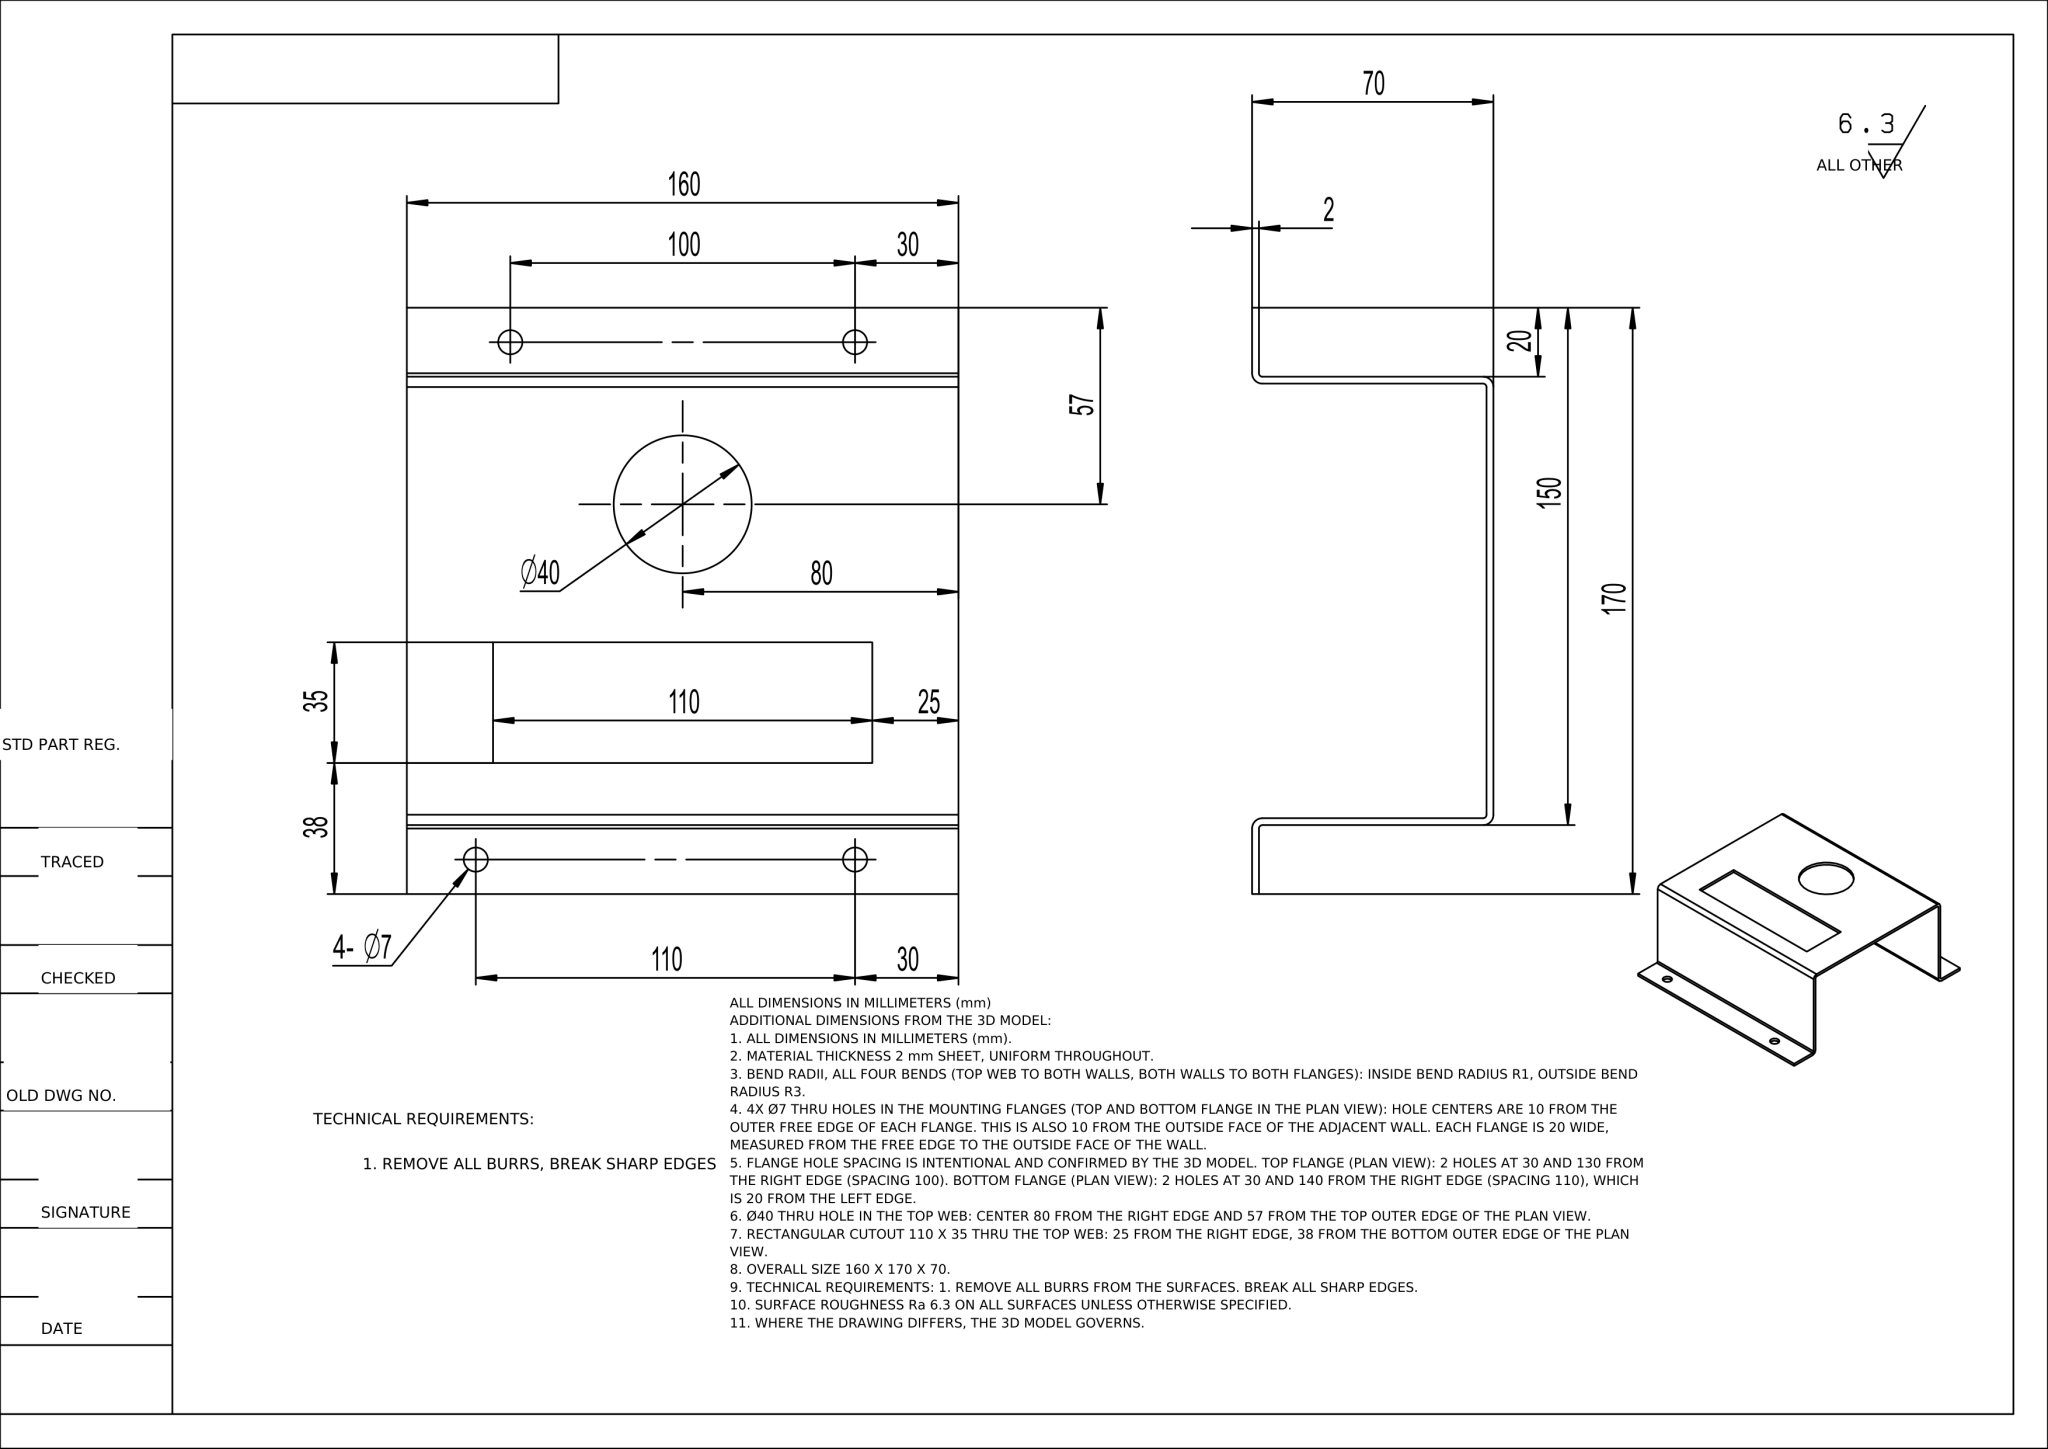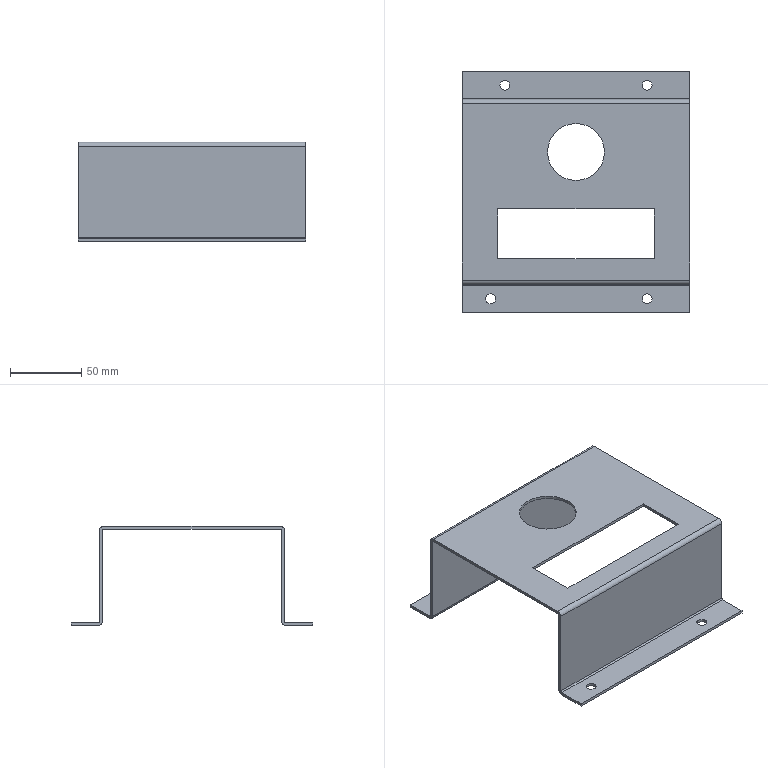Part | NX | mm | 1 solid | 31 faces | box 160 x 170 x 70 mm | volume 86300 mm3 | plane 18 | cylinder 13 | commonest cylinder face diameters 2 x4 6 x4 7 x4 40 x1
STEP:
#1=CARTESIAN_POINT('',(0.,0.,0.));
#2=DIRECTION('',(0.,0.,1.));
#3=DIRECTION('',(1.,0.,0.));
#4=AXIS2_PLACEMENT_3D('',#1,#2,#3);
#5=(LENGTH_UNIT()NAMED_UNIT(*)SI_UNIT(.MILLI.,.METRE.));
#6=UNCERTAINTY_MEASURE_WITH_UNIT(LENGTH_MEASURE(0.00002),#5,'','');
#7=(NAMED_UNIT(*)PLANE_ANGLE_UNIT()SI_UNIT($,.RADIAN.));
#8=PLANE_ANGLE_MEASURE_WITH_UNIT(PLANE_ANGLE_MEASURE(0.01745),#7);
#9=DIMENSIONAL_EXPONENTS(0.,0.,0.,0.,0.,0.,0.);
#10=(CONVERSION_BASED_UNIT('',#8)NAMED_UNIT(#9)PLANE_ANGLE_UNIT());
#11=(NAMED_UNIT(*)SI_UNIT($,.STERADIAN.)SOLID_ANGLE_UNIT());
#12=(GEOMETRIC_REPRESENTATION_CONTEXT(3)GLOBAL_UNCERTAINTY_ASSIGNED_CONTEXT((#6))GLOBAL_UNIT_ASSIGNED_CONTEXT((#5,#10,#11))REPRESENTATION_CONTEXT('',''));
#13=SHAPE_REPRESENTATION('',(#4),#12);
#14=CARTESIAN_POINT('',(25.,38.,68.));
#15=VERTEX_POINT('',#14);
#16=CARTESIAN_POINT('',(135.,38.,68.));
#17=VERTEX_POINT('',#16);
#18=CARTESIAN_POINT('',(25.,38.,68.));
#19=DIRECTION('',(1.,0.,0.));
#20=VECTOR('',#19,1.);
#21=LINE('',#18,#20);
#22=EDGE_CURVE('',#15,#17,#21,.T.);
#23=ORIENTED_EDGE('',*,*,#22,.F.);
#24=CARTESIAN_POINT('',(25.,73.,68.));
#25=VERTEX_POINT('',#24);
#26=CARTESIAN_POINT('',(25.,73.,68.));
#27=DIRECTION('',(0.,-1.,0.));
#28=VECTOR('',#27,1.);
#29=LINE('',#26,#28);
#30=EDGE_CURVE('',#25,#15,#29,.T.);
#31=ORIENTED_EDGE('',*,*,#30,.F.);
#32=CARTESIAN_POINT('',(135.,73.,68.));
#33=VERTEX_POINT('',#32);
#34=CARTESIAN_POINT('',(135.,73.,68.));
#35=DIRECTION('',(-1.,-0.,0.));
#36=VECTOR('',#35,1.);
#37=LINE('',#34,#36);
#38=EDGE_CURVE('',#33,#25,#37,.T.);
#39=ORIENTED_EDGE('',*,*,#38,.F.);
#40=CARTESIAN_POINT('',(135.,38.,68.));
#41=DIRECTION('',(0.,1.,0.));
#42=VECTOR('',#41,1.);
#43=LINE('',#40,#42);
#44=EDGE_CURVE('',#17,#33,#43,.T.);
#45=ORIENTED_EDGE('',*,*,#44,.F.);
#46=EDGE_LOOP('',(#23,#31,#39,#45));
#47=FACE_BOUND('',#46,.T.);
#48=CARTESIAN_POINT('',(160.,23.,68.));
#49=VERTEX_POINT('',#48);
#50=CARTESIAN_POINT('',(160.,147.,68.));
#51=VERTEX_POINT('',#50);
#52=CARTESIAN_POINT('',(160.,20.,68.));
#53=DIRECTION('',(0.,1.,0.));
#54=VECTOR('',#53,1.);
#55=LINE('',#52,#54);
#56=EDGE_CURVE('',#49,#51,#55,.T.);
#57=ORIENTED_EDGE('',*,*,#56,.T.);
#58=CARTESIAN_POINT('',(0.,147.,68.));
#59=VERTEX_POINT('',#58);
#60=CARTESIAN_POINT('',(0.,147.,68.));
#61=DIRECTION('',(1.,0.,0.));
#62=VECTOR('',#61,1.);
#63=LINE('',#60,#62);
#64=EDGE_CURVE('',#59,#51,#63,.T.);
#65=ORIENTED_EDGE('',*,*,#64,.F.);
#66=CARTESIAN_POINT('',(0.,23.,68.));
#67=VERTEX_POINT('',#66);
#68=CARTESIAN_POINT('',(0.,20.,68.));
#69=DIRECTION('',(0.,1.,0.));
#70=VECTOR('',#69,1.);
#71=LINE('',#68,#70);
#72=EDGE_CURVE('',#67,#59,#71,.T.);
#73=ORIENTED_EDGE('',*,*,#72,.F.);
#74=CARTESIAN_POINT('',(0.,23.,68.));
#75=DIRECTION('',(1.,0.,0.));
#76=VECTOR('',#75,1.);
#77=LINE('',#74,#76);
#78=EDGE_CURVE('',#67,#49,#77,.T.);
#79=ORIENTED_EDGE('',*,*,#78,.T.);
#80=EDGE_LOOP('',(#57,#65,#73,#79));
#81=FACE_BOUND('',#80,.T.);
#82=CARTESIAN_POINT('',(60.,113.,68.));
#83=VERTEX_POINT('',#82);
#84=CARTESIAN_POINT('',(80.,113.,68.));
#85=DIRECTION('',(0.,0.,1.));
#86=DIRECTION('',(-1.,0.,0.));
#87=AXIS2_PLACEMENT_3D('',#84,#85,#86);
#88=CIRCLE('',#87,20.);
#89=EDGE_CURVE('',#83,#83,#88,.T.);
#90=ORIENTED_EDGE('',*,*,#89,.F.);
#91=EDGE_LOOP('',(#90));
#92=FACE_BOUND('',#91,.T.);
#93=CARTESIAN_POINT('',(0.,20.,68.));
#94=DIRECTION('',(0.,0.,-1.));
#95=DIRECTION('',(-1.,0.,0.));
#96=AXIS2_PLACEMENT_3D('',#93,#94,#95);
#97=PLANE('',#96);
#98=ADVANCED_FACE('',(#47,#81,#92),#97,.F.);
#99=CARTESIAN_POINT('',(160.,170.,-2.));
#100=VERTEX_POINT('',#99);
#101=CARTESIAN_POINT('',(160.,170.,0.));
#102=VERTEX_POINT('',#101);
#103=CARTESIAN_POINT('',(160.,170.,0.));
#104=DIRECTION('',(0.,0.,1.));
#105=VECTOR('',#104,1.);
#106=LINE('',#103,#105);
#107=EDGE_CURVE('',#100,#102,#106,.T.);
#108=ORIENTED_EDGE('',*,*,#107,.F.);
#109=CARTESIAN_POINT('',(0.,170.,-2.));
#110=VERTEX_POINT('',#109);
#111=CARTESIAN_POINT('',(0.,170.,-2.));
#112=DIRECTION('',(1.,0.,0.));
#113=VECTOR('',#112,1.);
#114=LINE('',#111,#113);
#115=EDGE_CURVE('',#110,#100,#114,.T.);
#116=ORIENTED_EDGE('',*,*,#115,.F.);
#117=CARTESIAN_POINT('',(0.,170.,0.));
#118=VERTEX_POINT('',#117);
#119=CARTESIAN_POINT('',(0.,170.,0.));
#120=DIRECTION('',(0.,0.,1.));
#121=VECTOR('',#120,1.);
#122=LINE('',#119,#121);
#123=EDGE_CURVE('',#110,#118,#122,.T.);
#124=ORIENTED_EDGE('',*,*,#123,.T.);
#125=CARTESIAN_POINT('',(0.,170.,0.));
#126=DIRECTION('',(1.,0.,0.));
#127=VECTOR('',#126,1.);
#128=LINE('',#125,#127);
#129=EDGE_CURVE('',#118,#102,#128,.T.);
#130=ORIENTED_EDGE('',*,*,#129,.T.);
#131=EDGE_LOOP('',(#108,#116,#124,#130));
#132=FACE_OUTER_BOUND('',#131,.T.);
#133=CARTESIAN_POINT('',(0.,170.,0.));
#134=DIRECTION('',(0.,1.,0.));
#135=DIRECTION('',(1.,0.,0.));
#136=AXIS2_PLACEMENT_3D('',#133,#134,#135);
#137=PLANE('',#136);
#138=ADVANCED_FACE('',(#132),#137,.T.);
#139=CARTESIAN_POINT('',(0.,0.,0.));
#140=VERTEX_POINT('',#139);
#141=CARTESIAN_POINT('',(0.,19.,0.));
#142=VERTEX_POINT('',#141);
#143=CARTESIAN_POINT('',(0.,0.,0.));
#144=DIRECTION('',(0.,1.,0.));
#145=VECTOR('',#144,1.);
#146=LINE('',#143,#145);
#147=EDGE_CURVE('',#140,#142,#146,.T.);
#148=ORIENTED_EDGE('',*,*,#147,.T.);
#149=CARTESIAN_POINT('',(0.,20.,1.));
#150=VERTEX_POINT('',#149);
#151=CARTESIAN_POINT('',(0.,19.,1.));
#152=DIRECTION('',(1.,0.,0.));
#153=DIRECTION('',(0.,0.,1.));
#154=AXIS2_PLACEMENT_3D('',#151,#152,#153);
#155=CIRCLE('',#154,1.);
#156=EDGE_CURVE('',#142,#150,#155,.T.);
#157=ORIENTED_EDGE('',*,*,#156,.T.);
#158=CARTESIAN_POINT('',(0.,20.,65.));
#159=VERTEX_POINT('',#158);
#160=CARTESIAN_POINT('',(0.,20.,0.));
#161=DIRECTION('',(0.,0.,1.));
#162=VECTOR('',#161,1.);
#163=LINE('',#160,#162);
#164=EDGE_CURVE('',#150,#159,#163,.T.);
#165=ORIENTED_EDGE('',*,*,#164,.T.);
#166=CARTESIAN_POINT('',(0.,23.,65.));
#167=DIRECTION('',(-1.,0.,0.));
#168=DIRECTION('',(0.,0.,-1.));
#169=AXIS2_PLACEMENT_3D('',#166,#167,#168);
#170=CIRCLE('',#169,3.);
#171=EDGE_CURVE('',#159,#67,#170,.T.);
#172=ORIENTED_EDGE('',*,*,#171,.T.);
#173=ORIENTED_EDGE('',*,*,#72,.T.);
#174=CARTESIAN_POINT('',(0.,150.,65.));
#175=VERTEX_POINT('',#174);
#176=CARTESIAN_POINT('',(0.,147.,65.));
#177=DIRECTION('',(-1.,0.,0.));
#178=DIRECTION('',(0.,0.,-1.));
#179=AXIS2_PLACEMENT_3D('',#176,#177,#178);
#180=CIRCLE('',#179,3.);
#181=EDGE_CURVE('',#59,#175,#180,.T.);
#182=ORIENTED_EDGE('',*,*,#181,.T.);
#183=CARTESIAN_POINT('',(0.,150.,1.));
#184=VERTEX_POINT('',#183);
#185=CARTESIAN_POINT('',(0.,150.,68.));
#186=DIRECTION('',(0.,0.,-1.));
#187=VECTOR('',#186,1.);
#188=LINE('',#185,#187);
#189=EDGE_CURVE('',#175,#184,#188,.T.);
#190=ORIENTED_EDGE('',*,*,#189,.T.);
#191=CARTESIAN_POINT('',(0.,151.,0.));
#192=VERTEX_POINT('',#191);
#193=CARTESIAN_POINT('',(0.,151.,1.));
#194=DIRECTION('',(1.,0.,0.));
#195=DIRECTION('',(0.,0.,1.));
#196=AXIS2_PLACEMENT_3D('',#193,#194,#195);
#197=CIRCLE('',#196,1.);
#198=EDGE_CURVE('',#184,#192,#197,.T.);
#199=ORIENTED_EDGE('',*,*,#198,.T.);
#200=CARTESIAN_POINT('',(0.,150.,0.));
#201=DIRECTION('',(0.,1.,0.));
#202=VECTOR('',#201,1.);
#203=LINE('',#200,#202);
#204=EDGE_CURVE('',#192,#118,#203,.T.);
#205=ORIENTED_EDGE('',*,*,#204,.T.);
#206=ORIENTED_EDGE('',*,*,#123,.F.);
#207=CARTESIAN_POINT('',(0.,151.,-2.));
#208=VERTEX_POINT('',#207);
#209=CARTESIAN_POINT('',(0.,150.,-2.));
#210=DIRECTION('',(0.,1.,0.));
#211=VECTOR('',#210,1.);
#212=LINE('',#209,#211);
#213=EDGE_CURVE('',#208,#110,#212,.T.);
#214=ORIENTED_EDGE('',*,*,#213,.F.);
#215=CARTESIAN_POINT('',(0.,148.,1.));
#216=VERTEX_POINT('',#215);
#217=CARTESIAN_POINT('',(0.,151.,1.));
#218=DIRECTION('',(1.,0.,0.));
#219=DIRECTION('',(0.,0.,-1.));
#220=AXIS2_PLACEMENT_3D('',#217,#218,#219);
#221=CIRCLE('',#220,3.);
#222=EDGE_CURVE('',#216,#208,#221,.T.);
#223=ORIENTED_EDGE('',*,*,#222,.F.);
#224=CARTESIAN_POINT('',(0.,148.,65.));
#225=VERTEX_POINT('',#224);
#226=CARTESIAN_POINT('',(0.,148.,68.));
#227=DIRECTION('',(0.,0.,-1.));
#228=VECTOR('',#227,1.);
#229=LINE('',#226,#228);
#230=EDGE_CURVE('',#225,#216,#229,.T.);
#231=ORIENTED_EDGE('',*,*,#230,.F.);
#232=CARTESIAN_POINT('',(0.,147.,66.));
#233=VERTEX_POINT('',#232);
#234=CARTESIAN_POINT('',(0.,147.,65.));
#235=DIRECTION('',(-1.,0.,0.));
#236=DIRECTION('',(0.,0.,-1.));
#237=AXIS2_PLACEMENT_3D('',#234,#235,#236);
#238=CIRCLE('',#237,1.);
#239=EDGE_CURVE('',#233,#225,#238,.T.);
#240=ORIENTED_EDGE('',*,*,#239,.F.);
#241=CARTESIAN_POINT('',(0.,23.,66.));
#242=VERTEX_POINT('',#241);
#243=CARTESIAN_POINT('',(0.,20.,66.));
#244=DIRECTION('',(0.,1.,0.));
#245=VECTOR('',#244,1.);
#246=LINE('',#243,#245);
#247=EDGE_CURVE('',#242,#233,#246,.T.);
#248=ORIENTED_EDGE('',*,*,#247,.F.);
#249=CARTESIAN_POINT('',(0.,22.,65.));
#250=VERTEX_POINT('',#249);
#251=CARTESIAN_POINT('',(0.,23.,65.));
#252=DIRECTION('',(-1.,0.,0.));
#253=DIRECTION('',(0.,0.,-1.));
#254=AXIS2_PLACEMENT_3D('',#251,#252,#253);
#255=CIRCLE('',#254,1.);
#256=EDGE_CURVE('',#250,#242,#255,.T.);
#257=ORIENTED_EDGE('',*,*,#256,.F.);
#258=CARTESIAN_POINT('',(0.,22.,1.));
#259=VERTEX_POINT('',#258);
#260=CARTESIAN_POINT('',(0.,22.,-0.));
#261=DIRECTION('',(0.,0.,1.));
#262=VECTOR('',#261,1.);
#263=LINE('',#260,#262);
#264=EDGE_CURVE('',#259,#250,#263,.T.);
#265=ORIENTED_EDGE('',*,*,#264,.F.);
#266=CARTESIAN_POINT('',(0.,19.,-2.));
#267=VERTEX_POINT('',#266);
#268=CARTESIAN_POINT('',(0.,19.,1.));
#269=DIRECTION('',(1.,0.,0.));
#270=DIRECTION('',(0.,0.,-1.));
#271=AXIS2_PLACEMENT_3D('',#268,#269,#270);
#272=CIRCLE('',#271,3.);
#273=EDGE_CURVE('',#267,#259,#272,.T.);
#274=ORIENTED_EDGE('',*,*,#273,.F.);
#275=CARTESIAN_POINT('',(0.,0.,-2.));
#276=VERTEX_POINT('',#275);
#277=CARTESIAN_POINT('',(0.,0.,-2.));
#278=DIRECTION('',(0.,1.,0.));
#279=VECTOR('',#278,1.);
#280=LINE('',#277,#279);
#281=EDGE_CURVE('',#276,#267,#280,.T.);
#282=ORIENTED_EDGE('',*,*,#281,.F.);
#283=CARTESIAN_POINT('',(0.,0.,0.));
#284=DIRECTION('',(0.,0.,1.));
#285=VECTOR('',#284,1.);
#286=LINE('',#283,#285);
#287=EDGE_CURVE('',#276,#140,#286,.T.);
#288=ORIENTED_EDGE('',*,*,#287,.T.);
#289=EDGE_LOOP('',(#148,#157,#165,#172,#173,#182,#190,#199,#205,#206,#214,#223,#231,#240,#248,#257,#265,#274,#282,#288));
#290=FACE_OUTER_BOUND('',#289,.T.);
#291=CARTESIAN_POINT('',(0.,0.,0.));
#292=DIRECTION('',(-1.,0.,0.));
#293=DIRECTION('',(0.,1.,0.));
#294=AXIS2_PLACEMENT_3D('',#291,#292,#293);
#295=PLANE('',#294);
#296=ADVANCED_FACE('',(#290),#295,.T.);
#297=ORIENTED_EDGE('',*,*,#287,.F.);
#298=CARTESIAN_POINT('',(160.,0.,-2.));
#299=VERTEX_POINT('',#298);
#300=CARTESIAN_POINT('',(0.,0.,-2.));
#301=DIRECTION('',(1.,0.,0.));
#302=VECTOR('',#301,1.);
#303=LINE('',#300,#302);
#304=EDGE_CURVE('',#276,#299,#303,.T.);
#305=ORIENTED_EDGE('',*,*,#304,.T.);
#306=CARTESIAN_POINT('',(160.,0.,0.));
#307=VERTEX_POINT('',#306);
#308=CARTESIAN_POINT('',(160.,0.,0.));
#309=DIRECTION('',(0.,0.,1.));
#310=VECTOR('',#309,1.);
#311=LINE('',#308,#310);
#312=EDGE_CURVE('',#299,#307,#311,.T.);
#313=ORIENTED_EDGE('',*,*,#312,.T.);
#314=CARTESIAN_POINT('',(0.,0.,0.));
#315=DIRECTION('',(1.,0.,0.));
#316=VECTOR('',#315,1.);
#317=LINE('',#314,#316);
#318=EDGE_CURVE('',#140,#307,#317,.T.);
#319=ORIENTED_EDGE('',*,*,#318,.F.);
#320=EDGE_LOOP('',(#297,#305,#313,#319));
#321=FACE_OUTER_BOUND('',#320,.T.);
#322=CARTESIAN_POINT('',(0.,0.,0.));
#323=DIRECTION('',(0.,1.,0.));
#324=DIRECTION('',(1.,0.,0.));
#325=AXIS2_PLACEMENT_3D('',#322,#323,#324);
#326=PLANE('',#325);
#327=ADVANCED_FACE('',(#321),#326,.F.);
#328=CARTESIAN_POINT('',(160.,19.,-2.));
#329=VERTEX_POINT('',#328);
#330=CARTESIAN_POINT('',(160.,22.,1.));
#331=VERTEX_POINT('',#330);
#332=CARTESIAN_POINT('',(160.,19.,1.));
#333=DIRECTION('',(1.,0.,0.));
#334=DIRECTION('',(0.,0.,-1.));
#335=AXIS2_PLACEMENT_3D('',#332,#333,#334);
#336=CIRCLE('',#335,3.);
#337=EDGE_CURVE('',#329,#331,#336,.T.);
#338=ORIENTED_EDGE('',*,*,#337,.T.);
#339=CARTESIAN_POINT('',(160.,22.,65.));
#340=VERTEX_POINT('',#339);
#341=CARTESIAN_POINT('',(160.,22.,-0.));
#342=DIRECTION('',(0.,0.,1.));
#343=VECTOR('',#342,1.);
#344=LINE('',#341,#343);
#345=EDGE_CURVE('',#331,#340,#344,.T.);
#346=ORIENTED_EDGE('',*,*,#345,.T.);
#347=CARTESIAN_POINT('',(160.,23.,66.));
#348=VERTEX_POINT('',#347);
#349=CARTESIAN_POINT('',(160.,23.,65.));
#350=DIRECTION('',(-1.,0.,0.));
#351=DIRECTION('',(0.,0.,-1.));
#352=AXIS2_PLACEMENT_3D('',#349,#350,#351);
#353=CIRCLE('',#352,1.);
#354=EDGE_CURVE('',#340,#348,#353,.T.);
#355=ORIENTED_EDGE('',*,*,#354,.T.);
#356=CARTESIAN_POINT('',(160.,147.,66.));
#357=VERTEX_POINT('',#356);
#358=CARTESIAN_POINT('',(160.,20.,66.));
#359=DIRECTION('',(0.,1.,0.));
#360=VECTOR('',#359,1.);
#361=LINE('',#358,#360);
#362=EDGE_CURVE('',#348,#357,#361,.T.);
#363=ORIENTED_EDGE('',*,*,#362,.T.);
#364=CARTESIAN_POINT('',(160.,148.,65.));
#365=VERTEX_POINT('',#364);
#366=CARTESIAN_POINT('',(160.,147.,65.));
#367=DIRECTION('',(-1.,0.,0.));
#368=DIRECTION('',(0.,0.,-1.));
#369=AXIS2_PLACEMENT_3D('',#366,#367,#368);
#370=CIRCLE('',#369,1.);
#371=EDGE_CURVE('',#357,#365,#370,.T.);
#372=ORIENTED_EDGE('',*,*,#371,.T.);
#373=CARTESIAN_POINT('',(160.,148.,1.));
#374=VERTEX_POINT('',#373);
#375=CARTESIAN_POINT('',(160.,148.,68.));
#376=DIRECTION('',(0.,0.,-1.));
#377=VECTOR('',#376,1.);
#378=LINE('',#375,#377);
#379=EDGE_CURVE('',#365,#374,#378,.T.);
#380=ORIENTED_EDGE('',*,*,#379,.T.);
#381=CARTESIAN_POINT('',(160.,151.,-2.));
#382=VERTEX_POINT('',#381);
#383=CARTESIAN_POINT('',(160.,151.,1.));
#384=DIRECTION('',(1.,0.,0.));
#385=DIRECTION('',(0.,0.,-1.));
#386=AXIS2_PLACEMENT_3D('',#383,#384,#385);
#387=CIRCLE('',#386,3.);
#388=EDGE_CURVE('',#374,#382,#387,.T.);
#389=ORIENTED_EDGE('',*,*,#388,.T.);
#390=CARTESIAN_POINT('',(160.,150.,-2.));
#391=DIRECTION('',(0.,1.,0.));
#392=VECTOR('',#391,1.);
#393=LINE('',#390,#392);
#394=EDGE_CURVE('',#382,#100,#393,.T.);
#395=ORIENTED_EDGE('',*,*,#394,.T.);
#396=ORIENTED_EDGE('',*,*,#107,.T.);
#397=CARTESIAN_POINT('',(160.,151.,0.));
#398=VERTEX_POINT('',#397);
#399=CARTESIAN_POINT('',(160.,150.,0.));
#400=DIRECTION('',(0.,1.,0.));
#401=VECTOR('',#400,1.);
#402=LINE('',#399,#401);
#403=EDGE_CURVE('',#398,#102,#402,.T.);
#404=ORIENTED_EDGE('',*,*,#403,.F.);
#405=CARTESIAN_POINT('',(160.,150.,1.));
#406=VERTEX_POINT('',#405);
#407=CARTESIAN_POINT('',(160.,151.,1.));
#408=DIRECTION('',(1.,0.,0.));
#409=DIRECTION('',(0.,0.,1.));
#410=AXIS2_PLACEMENT_3D('',#407,#408,#409);
#411=CIRCLE('',#410,1.);
#412=EDGE_CURVE('',#406,#398,#411,.T.);
#413=ORIENTED_EDGE('',*,*,#412,.F.);
#414=CARTESIAN_POINT('',(160.,150.,65.));
#415=VERTEX_POINT('',#414);
#416=CARTESIAN_POINT('',(160.,150.,68.));
#417=DIRECTION('',(0.,0.,-1.));
#418=VECTOR('',#417,1.);
#419=LINE('',#416,#418);
#420=EDGE_CURVE('',#415,#406,#419,.T.);
#421=ORIENTED_EDGE('',*,*,#420,.F.);
#422=CARTESIAN_POINT('',(160.,147.,65.));
#423=DIRECTION('',(-1.,0.,0.));
#424=DIRECTION('',(0.,0.,-1.));
#425=AXIS2_PLACEMENT_3D('',#422,#423,#424);
#426=CIRCLE('',#425,3.);
#427=EDGE_CURVE('',#51,#415,#426,.T.);
#428=ORIENTED_EDGE('',*,*,#427,.F.);
#429=ORIENTED_EDGE('',*,*,#56,.F.);
#430=CARTESIAN_POINT('',(160.,20.,65.));
#431=VERTEX_POINT('',#430);
#432=CARTESIAN_POINT('',(160.,23.,65.));
#433=DIRECTION('',(-1.,0.,0.));
#434=DIRECTION('',(0.,0.,-1.));
#435=AXIS2_PLACEMENT_3D('',#432,#433,#434);
#436=CIRCLE('',#435,3.);
#437=EDGE_CURVE('',#431,#49,#436,.T.);
#438=ORIENTED_EDGE('',*,*,#437,.F.);
#439=CARTESIAN_POINT('',(160.,20.,1.));
#440=VERTEX_POINT('',#439);
#441=CARTESIAN_POINT('',(160.,20.,0.));
#442=DIRECTION('',(0.,0.,1.));
#443=VECTOR('',#442,1.);
#444=LINE('',#441,#443);
#445=EDGE_CURVE('',#440,#431,#444,.T.);
#446=ORIENTED_EDGE('',*,*,#445,.F.);
#447=CARTESIAN_POINT('',(160.,19.,0.));
#448=VERTEX_POINT('',#447);
#449=CARTESIAN_POINT('',(160.,19.,1.));
#450=DIRECTION('',(1.,0.,0.));
#451=DIRECTION('',(0.,0.,1.));
#452=AXIS2_PLACEMENT_3D('',#449,#450,#451);
#453=CIRCLE('',#452,1.);
#454=EDGE_CURVE('',#448,#440,#453,.T.);
#455=ORIENTED_EDGE('',*,*,#454,.F.);
#456=CARTESIAN_POINT('',(160.,0.,0.));
#457=DIRECTION('',(0.,1.,0.));
#458=VECTOR('',#457,1.);
#459=LINE('',#456,#458);
#460=EDGE_CURVE('',#307,#448,#459,.T.);
#461=ORIENTED_EDGE('',*,*,#460,.F.);
#462=ORIENTED_EDGE('',*,*,#312,.F.);
#463=CARTESIAN_POINT('',(160.,0.,-2.));
#464=DIRECTION('',(0.,1.,0.));
#465=VECTOR('',#464,1.);
#466=LINE('',#463,#465);
#467=EDGE_CURVE('',#299,#329,#466,.T.);
#468=ORIENTED_EDGE('',*,*,#467,.T.);
#469=EDGE_LOOP('',(#338,#346,#355,#363,#372,#380,#389,#395,#396,#404,#413,#421,#428,#429,#438,#446,#455,#461,#462,#468));
#470=FACE_OUTER_BOUND('',#469,.T.);
#471=CARTESIAN_POINT('',(160.,19.,1.));
#472=DIRECTION('',(1.,0.,0.));
#473=DIRECTION('',(0.,0.,-1.));
#474=AXIS2_PLACEMENT_3D('',#471,#472,#473);
#475=PLANE('',#474);
#476=ADVANCED_FACE('',(#470),#475,.T.);
#477=CARTESIAN_POINT('',(126.5,10.,0.));
#478=VERTEX_POINT('',#477);
#479=CARTESIAN_POINT('',(130.,10.,0.));
#480=DIRECTION('',(0.,0.,-1.));
#481=DIRECTION('',(-1.,0.,0.));
#482=AXIS2_PLACEMENT_3D('',#479,#480,#481);
#483=CIRCLE('',#482,3.5);
#484=EDGE_CURVE('',#478,#478,#483,.T.);
#485=ORIENTED_EDGE('',*,*,#484,.T.);
#486=EDGE_LOOP('',(#485));
#487=FACE_BOUND('',#486,.T.);
#488=CARTESIAN_POINT('',(16.5,10.,0.));
#489=VERTEX_POINT('',#488);
#490=CARTESIAN_POINT('',(20.,10.,0.));
#491=DIRECTION('',(0.,0.,-1.));
#492=DIRECTION('',(-1.,0.,0.));
#493=AXIS2_PLACEMENT_3D('',#490,#491,#492);
#494=CIRCLE('',#493,3.5);
#495=EDGE_CURVE('',#489,#489,#494,.T.);
#496=ORIENTED_EDGE('',*,*,#495,.T.);
#497=EDGE_LOOP('',(#496));
#498=FACE_BOUND('',#497,.T.);
#499=ORIENTED_EDGE('',*,*,#460,.T.);
#500=CARTESIAN_POINT('',(0.,19.,0.));
#501=DIRECTION('',(1.,0.,0.));
#502=VECTOR('',#501,1.);
#503=LINE('',#500,#502);
#504=EDGE_CURVE('',#142,#448,#503,.T.);
#505=ORIENTED_EDGE('',*,*,#504,.F.);
#506=ORIENTED_EDGE('',*,*,#147,.F.);
#507=ORIENTED_EDGE('',*,*,#318,.T.);
#508=EDGE_LOOP('',(#499,#505,#506,#507));
#509=FACE_BOUND('',#508,.T.);
#510=CARTESIAN_POINT('',(0.,0.,0.));
#511=DIRECTION('',(0.,0.,-1.));
#512=DIRECTION('',(-1.,0.,0.));
#513=AXIS2_PLACEMENT_3D('',#510,#511,#512);
#514=PLANE('',#513);
#515=ADVANCED_FACE('',(#487,#498,#509),#514,.F.);
#516=ORIENTED_EDGE('',*,*,#454,.T.);
#517=CARTESIAN_POINT('',(0.,20.,1.));
#518=DIRECTION('',(1.,0.,0.));
#519=VECTOR('',#518,1.);
#520=LINE('',#517,#519);
#521=EDGE_CURVE('',#150,#440,#520,.T.);
#522=ORIENTED_EDGE('',*,*,#521,.F.);
#523=ORIENTED_EDGE('',*,*,#156,.F.);
#524=ORIENTED_EDGE('',*,*,#504,.T.);
#525=EDGE_LOOP('',(#516,#522,#523,#524));
#526=FACE_OUTER_BOUND('',#525,.T.);
#527=CARTESIAN_POINT('',(0.,19.,1.));
#528=DIRECTION('',(1.,0.,0.));
#529=DIRECTION('',(0.,0.,-1.));
#530=AXIS2_PLACEMENT_3D('',#527,#528,#529);
#531=CYLINDRICAL_SURFACE('',#530,1.);
#532=ADVANCED_FACE('',(#526),#531,.F.);
#533=ORIENTED_EDGE('',*,*,#445,.T.);
#534=CARTESIAN_POINT('',(0.,20.,65.));
#535=DIRECTION('',(1.,0.,0.));
#536=VECTOR('',#535,1.);
#537=LINE('',#534,#536);
#538=EDGE_CURVE('',#159,#431,#537,.T.);
#539=ORIENTED_EDGE('',*,*,#538,.F.);
#540=ORIENTED_EDGE('',*,*,#164,.F.);
#541=ORIENTED_EDGE('',*,*,#521,.T.);
#542=EDGE_LOOP('',(#533,#539,#540,#541));
#543=FACE_OUTER_BOUND('',#542,.T.);
#544=CARTESIAN_POINT('',(0.,20.,0.));
#545=DIRECTION('',(0.,1.,-0.));
#546=DIRECTION('',(0.,0.,1.));
#547=AXIS2_PLACEMENT_3D('',#544,#545,#546);
#548=PLANE('',#547);
#549=ADVANCED_FACE('',(#543),#548,.F.);
#550=ORIENTED_EDGE('',*,*,#437,.T.);
#551=ORIENTED_EDGE('',*,*,#78,.F.);
#552=ORIENTED_EDGE('',*,*,#171,.F.);
#553=ORIENTED_EDGE('',*,*,#538,.T.);
#554=EDGE_LOOP('',(#550,#551,#552,#553));
#555=FACE_OUTER_BOUND('',#554,.T.);
#556=CARTESIAN_POINT('',(0.,23.,65.));
#557=DIRECTION('',(1.,0.,0.));
#558=DIRECTION('',(0.,0.,-1.));
#559=AXIS2_PLACEMENT_3D('',#556,#557,#558);
#560=CYLINDRICAL_SURFACE('',#559,3.);
#561=ADVANCED_FACE('',(#555),#560,.T.);
#562=ORIENTED_EDGE('',*,*,#427,.T.);
#563=CARTESIAN_POINT('',(0.,150.,65.));
#564=DIRECTION('',(1.,0.,0.));
#565=VECTOR('',#564,1.);
#566=LINE('',#563,#565);
#567=EDGE_CURVE('',#175,#415,#566,.T.);
#568=ORIENTED_EDGE('',*,*,#567,.F.);
#569=ORIENTED_EDGE('',*,*,#181,.F.);
#570=ORIENTED_EDGE('',*,*,#64,.T.);
#571=EDGE_LOOP('',(#562,#568,#569,#570));
#572=FACE_OUTER_BOUND('',#571,.T.);
#573=CARTESIAN_POINT('',(0.,147.,65.));
#574=DIRECTION('',(1.,0.,0.));
#575=DIRECTION('',(0.,0.,-1.));
#576=AXIS2_PLACEMENT_3D('',#573,#574,#575);
#577=CYLINDRICAL_SURFACE('',#576,3.);
#578=ADVANCED_FACE('',(#572),#577,.T.);
#579=ORIENTED_EDGE('',*,*,#420,.T.);
#580=CARTESIAN_POINT('',(0.,150.,1.));
#581=DIRECTION('',(1.,0.,0.));
#582=VECTOR('',#581,1.);
#583=LINE('',#580,#582);
#584=EDGE_CURVE('',#184,#406,#583,.T.);
#585=ORIENTED_EDGE('',*,*,#584,.F.);
#586=ORIENTED_EDGE('',*,*,#189,.F.);
#587=ORIENTED_EDGE('',*,*,#567,.T.);
#588=EDGE_LOOP('',(#579,#585,#586,#587));
#589=FACE_OUTER_BOUND('',#588,.T.);
#590=CARTESIAN_POINT('',(0.,150.,68.));
#591=DIRECTION('',(0.,-1.,0.));
#592=DIRECTION('',(0.,0.,-1.));
#593=AXIS2_PLACEMENT_3D('',#590,#591,#592);
#594=PLANE('',#593);
#595=ADVANCED_FACE('',(#589),#594,.F.);
#596=ORIENTED_EDGE('',*,*,#412,.T.);
#597=CARTESIAN_POINT('',(0.,151.,0.));
#598=DIRECTION('',(1.,0.,0.));
#599=VECTOR('',#598,1.);
#600=LINE('',#597,#599);
#601=EDGE_CURVE('',#192,#398,#600,.T.);
#602=ORIENTED_EDGE('',*,*,#601,.F.);
#603=ORIENTED_EDGE('',*,*,#198,.F.);
#604=ORIENTED_EDGE('',*,*,#584,.T.);
#605=EDGE_LOOP('',(#596,#602,#603,#604));
#606=FACE_OUTER_BOUND('',#605,.T.);
#607=CARTESIAN_POINT('',(0.,151.,1.));
#608=DIRECTION('',(1.,0.,0.));
#609=DIRECTION('',(0.,0.,-1.));
#610=AXIS2_PLACEMENT_3D('',#607,#608,#609);
#611=CYLINDRICAL_SURFACE('',#610,1.);
#612=ADVANCED_FACE('',(#606),#611,.F.);
#613=CARTESIAN_POINT('',(126.5,160.,0.));
#614=VERTEX_POINT('',#613);
#615=CARTESIAN_POINT('',(130.,160.,0.));
#616=DIRECTION('',(0.,0.,-1.));
#617=DIRECTION('',(-1.,0.,0.));
#618=AXIS2_PLACEMENT_3D('',#615,#616,#617);
#619=CIRCLE('',#618,3.5);
#620=EDGE_CURVE('',#614,#614,#619,.T.);
#621=ORIENTED_EDGE('',*,*,#620,.T.);
#622=EDGE_LOOP('',(#621));
#623=FACE_BOUND('',#622,.T.);
#624=CARTESIAN_POINT('',(26.5,160.,0.));
#625=VERTEX_POINT('',#624);
#626=CARTESIAN_POINT('',(30.,160.,0.));
#627=DIRECTION('',(0.,0.,-1.));
#628=DIRECTION('',(-1.,0.,0.));
#629=AXIS2_PLACEMENT_3D('',#626,#627,#628);
#630=CIRCLE('',#629,3.5);
#631=EDGE_CURVE('',#625,#625,#630,.T.);
#632=ORIENTED_EDGE('',*,*,#631,.T.);
#633=EDGE_LOOP('',(#632));
#634=FACE_BOUND('',#633,.T.);
#635=ORIENTED_EDGE('',*,*,#403,.T.);
#636=ORIENTED_EDGE('',*,*,#129,.F.);
#637=ORIENTED_EDGE('',*,*,#204,.F.);
#638=ORIENTED_EDGE('',*,*,#601,.T.);
#639=EDGE_LOOP('',(#635,#636,#637,#638));
#640=FACE_BOUND('',#639,.T.);
#641=CARTESIAN_POINT('',(0.,150.,0.));
#642=DIRECTION('',(0.,0.,-1.));
#643=DIRECTION('',(-1.,0.,0.));
#644=AXIS2_PLACEMENT_3D('',#641,#642,#643);
#645=PLANE('',#644);
#646=ADVANCED_FACE('',(#623,#634,#640),#645,.F.);
#647=CARTESIAN_POINT('',(126.5,10.,-2.));
#648=VERTEX_POINT('',#647);
#649=CARTESIAN_POINT('',(130.,10.,-2.));
#650=DIRECTION('',(0.,0.,-1.));
#651=DIRECTION('',(-1.,0.,0.));
#652=AXIS2_PLACEMENT_3D('',#649,#650,#651);
#653=CIRCLE('',#652,3.5);
#654=EDGE_CURVE('',#648,#648,#653,.T.);
#655=ORIENTED_EDGE('',*,*,#654,.F.);
#656=EDGE_LOOP('',(#655));
#657=FACE_BOUND('',#656,.T.);
#658=CARTESIAN_POINT('',(16.5,10.,-2.));
#659=VERTEX_POINT('',#658);
#660=CARTESIAN_POINT('',(20.,10.,-2.));
#661=DIRECTION('',(0.,0.,-1.));
#662=DIRECTION('',(-1.,0.,0.));
#663=AXIS2_PLACEMENT_3D('',#660,#661,#662);
#664=CIRCLE('',#663,3.5);
#665=EDGE_CURVE('',#659,#659,#664,.T.);
#666=ORIENTED_EDGE('',*,*,#665,.F.);
#667=EDGE_LOOP('',(#666));
#668=FACE_BOUND('',#667,.T.);
#669=ORIENTED_EDGE('',*,*,#467,.F.);
#670=ORIENTED_EDGE('',*,*,#304,.F.);
#671=ORIENTED_EDGE('',*,*,#281,.T.);
#672=CARTESIAN_POINT('',(0.,19.,-2.));
#673=DIRECTION('',(1.,0.,0.));
#674=VECTOR('',#673,1.);
#675=LINE('',#672,#674);
#676=EDGE_CURVE('',#267,#329,#675,.T.);
#677=ORIENTED_EDGE('',*,*,#676,.T.);
#678=EDGE_LOOP('',(#669,#670,#671,#677));
#679=FACE_BOUND('',#678,.T.);
#680=CARTESIAN_POINT('',(0.,0.,-2.));
#681=DIRECTION('',(0.,0.,-1.));
#682=DIRECTION('',(-1.,0.,0.));
#683=AXIS2_PLACEMENT_3D('',#680,#681,#682);
#684=PLANE('',#683);
#685=ADVANCED_FACE('',(#657,#668,#679),#684,.T.);
#686=ORIENTED_EDGE('',*,*,#337,.F.);
#687=ORIENTED_EDGE('',*,*,#676,.F.);
#688=ORIENTED_EDGE('',*,*,#273,.T.);
#689=CARTESIAN_POINT('',(0.,22.,1.));
#690=DIRECTION('',(1.,0.,0.));
#691=VECTOR('',#690,1.);
#692=LINE('',#689,#691);
#693=EDGE_CURVE('',#259,#331,#692,.T.);
#694=ORIENTED_EDGE('',*,*,#693,.T.);
#695=EDGE_LOOP('',(#686,#687,#688,#694));
#696=FACE_OUTER_BOUND('',#695,.T.);
#697=CARTESIAN_POINT('',(0.,19.,1.));
#698=DIRECTION('',(1.,0.,0.));
#699=DIRECTION('',(0.,0.,-1.));
#700=AXIS2_PLACEMENT_3D('',#697,#698,#699);
#701=CYLINDRICAL_SURFACE('',#700,3.);
#702=ADVANCED_FACE('',(#696),#701,.T.);
#703=ORIENTED_EDGE('',*,*,#345,.F.);
#704=ORIENTED_EDGE('',*,*,#693,.F.);
#705=ORIENTED_EDGE('',*,*,#264,.T.);
#706=CARTESIAN_POINT('',(0.,22.,65.));
#707=DIRECTION('',(1.,0.,0.));
#708=VECTOR('',#707,1.);
#709=LINE('',#706,#708);
#710=EDGE_CURVE('',#250,#340,#709,.T.);
#711=ORIENTED_EDGE('',*,*,#710,.T.);
#712=EDGE_LOOP('',(#703,#704,#705,#711));
#713=FACE_OUTER_BOUND('',#712,.T.);
#714=CARTESIAN_POINT('',(0.,22.,-0.));
#715=DIRECTION('',(0.,1.,-0.));
#716=DIRECTION('',(0.,0.,1.));
#717=AXIS2_PLACEMENT_3D('',#714,#715,#716);
#718=PLANE('',#717);
#719=ADVANCED_FACE('',(#713),#718,.T.);
#720=ORIENTED_EDGE('',*,*,#354,.F.);
#721=ORIENTED_EDGE('',*,*,#710,.F.);
#722=ORIENTED_EDGE('',*,*,#256,.T.);
#723=CARTESIAN_POINT('',(0.,23.,66.));
#724=DIRECTION('',(1.,0.,0.));
#725=VECTOR('',#724,1.);
#726=LINE('',#723,#725);
#727=EDGE_CURVE('',#242,#348,#726,.T.);
#728=ORIENTED_EDGE('',*,*,#727,.T.);
#729=EDGE_LOOP('',(#720,#721,#722,#728));
#730=FACE_OUTER_BOUND('',#729,.T.);
#731=CARTESIAN_POINT('',(0.,23.,65.));
#732=DIRECTION('',(1.,0.,0.));
#733=DIRECTION('',(0.,0.,-1.));
#734=AXIS2_PLACEMENT_3D('',#731,#732,#733);
#735=CYLINDRICAL_SURFACE('',#734,1.);
#736=ADVANCED_FACE('',(#730),#735,.F.);
#737=CARTESIAN_POINT('',(25.,38.,66.));
#738=VERTEX_POINT('',#737);
#739=CARTESIAN_POINT('',(25.,73.,66.));
#740=VERTEX_POINT('',#739);
#741=CARTESIAN_POINT('',(25.,20.,66.));
#742=DIRECTION('',(0.,1.,0.));
#743=VECTOR('',#742,1.);
#744=LINE('',#741,#743);
#745=EDGE_CURVE('',#738,#740,#744,.T.);
#746=ORIENTED_EDGE('',*,*,#745,.F.);
#747=CARTESIAN_POINT('',(135.,38.,66.));
#748=VERTEX_POINT('',#747);
#749=CARTESIAN_POINT('',(0.,38.,66.));
#750=DIRECTION('',(-1.,0.,0.));
#751=VECTOR('',#750,1.);
#752=LINE('',#749,#751);
#753=EDGE_CURVE('',#748,#738,#752,.T.);
#754=ORIENTED_EDGE('',*,*,#753,.F.);
#755=CARTESIAN_POINT('',(135.,73.,66.));
#756=VERTEX_POINT('',#755);
#757=CARTESIAN_POINT('',(135.,20.,66.));
#758=DIRECTION('',(0.,-1.,0.));
#759=VECTOR('',#758,1.);
#760=LINE('',#757,#759);
#761=EDGE_CURVE('',#756,#748,#760,.T.);
#762=ORIENTED_EDGE('',*,*,#761,.F.);
#763=CARTESIAN_POINT('',(-0.,73.,66.));
#764=DIRECTION('',(1.,0.,0.));
#765=VECTOR('',#764,1.);
#766=LINE('',#763,#765);
#767=EDGE_CURVE('',#740,#756,#766,.T.);
#768=ORIENTED_EDGE('',*,*,#767,.F.);
#769=EDGE_LOOP('',(#746,#754,#762,#768));
#770=FACE_BOUND('',#769,.T.);
#771=CARTESIAN_POINT('',(60.,113.,66.));
#772=VERTEX_POINT('',#771);
#773=CARTESIAN_POINT('',(80.,113.,66.));
#774=DIRECTION('',(0.,0.,-1.));
#775=DIRECTION('',(-1.,0.,0.));
#776=AXIS2_PLACEMENT_3D('',#773,#774,#775);
#777=CIRCLE('',#776,20.);
#778=EDGE_CURVE('',#772,#772,#777,.T.);
#779=ORIENTED_EDGE('',*,*,#778,.F.);
#780=EDGE_LOOP('',(#779));
#781=FACE_BOUND('',#780,.T.);
#782=ORIENTED_EDGE('',*,*,#362,.F.);
#783=ORIENTED_EDGE('',*,*,#727,.F.);
#784=ORIENTED_EDGE('',*,*,#247,.T.);
#785=CARTESIAN_POINT('',(0.,147.,66.));
#786=DIRECTION('',(1.,0.,0.));
#787=VECTOR('',#786,1.);
#788=LINE('',#785,#787);
#789=EDGE_CURVE('',#233,#357,#788,.T.);
#790=ORIENTED_EDGE('',*,*,#789,.T.);
#791=EDGE_LOOP('',(#782,#783,#784,#790));
#792=FACE_BOUND('',#791,.T.);
#793=CARTESIAN_POINT('',(0.,20.,66.));
#794=DIRECTION('',(0.,0.,-1.));
#795=DIRECTION('',(-1.,0.,0.));
#796=AXIS2_PLACEMENT_3D('',#793,#794,#795);
#797=PLANE('',#796);
#798=ADVANCED_FACE('',(#770,#781,#792),#797,.T.);
#799=ORIENTED_EDGE('',*,*,#371,.F.);
#800=ORIENTED_EDGE('',*,*,#789,.F.);
#801=ORIENTED_EDGE('',*,*,#239,.T.);
#802=CARTESIAN_POINT('',(0.,148.,65.));
#803=DIRECTION('',(1.,0.,0.));
#804=VECTOR('',#803,1.);
#805=LINE('',#802,#804);
#806=EDGE_CURVE('',#225,#365,#805,.T.);
#807=ORIENTED_EDGE('',*,*,#806,.T.);
#808=EDGE_LOOP('',(#799,#800,#801,#807));
#809=FACE_OUTER_BOUND('',#808,.T.);
#810=CARTESIAN_POINT('',(0.,147.,65.));
#811=DIRECTION('',(1.,0.,0.));
#812=DIRECTION('',(0.,0.,-1.));
#813=AXIS2_PLACEMENT_3D('',#810,#811,#812);
#814=CYLINDRICAL_SURFACE('',#813,1.);
#815=ADVANCED_FACE('',(#809),#814,.F.);
#816=ORIENTED_EDGE('',*,*,#379,.F.);
#817=ORIENTED_EDGE('',*,*,#806,.F.);
#818=ORIENTED_EDGE('',*,*,#230,.T.);
#819=CARTESIAN_POINT('',(0.,148.,1.));
#820=DIRECTION('',(1.,0.,0.));
#821=VECTOR('',#820,1.);
#822=LINE('',#819,#821);
#823=EDGE_CURVE('',#216,#374,#822,.T.);
#824=ORIENTED_EDGE('',*,*,#823,.T.);
#825=EDGE_LOOP('',(#816,#817,#818,#824));
#826=FACE_OUTER_BOUND('',#825,.T.);
#827=CARTESIAN_POINT('',(0.,148.,68.));
#828=DIRECTION('',(0.,-1.,0.));
#829=DIRECTION('',(0.,0.,-1.));
#830=AXIS2_PLACEMENT_3D('',#827,#828,#829);
#831=PLANE('',#830);
#832=ADVANCED_FACE('',(#826),#831,.T.);
#833=ORIENTED_EDGE('',*,*,#388,.F.);
#834=ORIENTED_EDGE('',*,*,#823,.F.);
#835=ORIENTED_EDGE('',*,*,#222,.T.);
#836=CARTESIAN_POINT('',(0.,151.,-2.));
#837=DIRECTION('',(1.,0.,0.));
#838=VECTOR('',#837,1.);
#839=LINE('',#836,#838);
#840=EDGE_CURVE('',#208,#382,#839,.T.);
#841=ORIENTED_EDGE('',*,*,#840,.T.);
#842=EDGE_LOOP('',(#833,#834,#835,#841));
#843=FACE_OUTER_BOUND('',#842,.T.);
#844=CARTESIAN_POINT('',(0.,151.,1.));
#845=DIRECTION('',(1.,0.,0.));
#846=DIRECTION('',(0.,0.,-1.));
#847=AXIS2_PLACEMENT_3D('',#844,#845,#846);
#848=CYLINDRICAL_SURFACE('',#847,3.);
#849=ADVANCED_FACE('',(#843),#848,.T.);
#850=CARTESIAN_POINT('',(126.5,160.,-2.));
#851=VERTEX_POINT('',#850);
#852=CARTESIAN_POINT('',(130.,160.,-2.));
#853=DIRECTION('',(0.,0.,-1.));
#854=DIRECTION('',(-1.,0.,0.));
#855=AXIS2_PLACEMENT_3D('',#852,#853,#854);
#856=CIRCLE('',#855,3.5);
#857=EDGE_CURVE('',#851,#851,#856,.T.);
#858=ORIENTED_EDGE('',*,*,#857,.F.);
#859=EDGE_LOOP('',(#858));
#860=FACE_BOUND('',#859,.T.);
#861=CARTESIAN_POINT('',(26.5,160.,-2.));
#862=VERTEX_POINT('',#861);
#863=CARTESIAN_POINT('',(30.,160.,-2.));
#864=DIRECTION('',(0.,0.,-1.));
#865=DIRECTION('',(-1.,0.,0.));
#866=AXIS2_PLACEMENT_3D('',#863,#864,#865);
#867=CIRCLE('',#866,3.5);
#868=EDGE_CURVE('',#862,#862,#867,.T.);
#869=ORIENTED_EDGE('',*,*,#868,.F.);
#870=EDGE_LOOP('',(#869));
#871=FACE_BOUND('',#870,.T.);
#872=ORIENTED_EDGE('',*,*,#394,.F.);
#873=ORIENTED_EDGE('',*,*,#840,.F.);
#874=ORIENTED_EDGE('',*,*,#213,.T.);
#875=ORIENTED_EDGE('',*,*,#115,.T.);
#876=EDGE_LOOP('',(#872,#873,#874,#875));
#877=FACE_BOUND('',#876,.T.);
#878=CARTESIAN_POINT('',(0.,150.,-2.));
#879=DIRECTION('',(0.,0.,-1.));
#880=DIRECTION('',(-1.,0.,0.));
#881=AXIS2_PLACEMENT_3D('',#878,#879,#880);
#882=PLANE('',#881);
#883=ADVANCED_FACE('',(#860,#871,#877),#882,.T.);
#884=ORIENTED_EDGE('',*,*,#778,.T.);
#885=EDGE_LOOP('',(#884));
#886=FACE_BOUND('',#885,.T.);
#887=ORIENTED_EDGE('',*,*,#89,.T.);
#888=EDGE_LOOP('',(#887));
#889=FACE_BOUND('',#888,.T.);
#890=CARTESIAN_POINT('',(80.,113.,56.));
#891=DIRECTION('',(0.,0.,1.));
#892=DIRECTION('',(1.,0.,0.));
#893=AXIS2_PLACEMENT_3D('',#890,#891,#892);
#894=CYLINDRICAL_SURFACE('',#893,20.);
#895=ADVANCED_FACE('',(#886,#889),#894,.F.);
#896=ORIENTED_EDGE('',*,*,#745,.T.);
#897=CARTESIAN_POINT('',(25.,73.,56.));
#898=DIRECTION('',(0.,0.,-1.));
#899=VECTOR('',#898,1.);
#900=LINE('',#897,#899);
#901=EDGE_CURVE('',#25,#740,#900,.T.);
#902=ORIENTED_EDGE('',*,*,#901,.F.);
#903=ORIENTED_EDGE('',*,*,#30,.T.);
#904=CARTESIAN_POINT('',(25.,38.,56.));
#905=DIRECTION('',(0.,0.,-1.));
#906=VECTOR('',#905,1.);
#907=LINE('',#904,#906);
#908=EDGE_CURVE('',#15,#738,#907,.T.);
#909=ORIENTED_EDGE('',*,*,#908,.T.);
#910=EDGE_LOOP('',(#896,#902,#903,#909));
#911=FACE_OUTER_BOUND('',#910,.T.);
#912=CARTESIAN_POINT('',(25.,73.,56.));
#913=DIRECTION('',(-1.,0.,0.));
#914=DIRECTION('',(0.,0.,1.));
#915=AXIS2_PLACEMENT_3D('',#912,#913,#914);
#916=PLANE('',#915);
#917=ADVANCED_FACE('',(#911),#916,.F.);
#918=ORIENTED_EDGE('',*,*,#753,.T.);
#919=ORIENTED_EDGE('',*,*,#908,.F.);
#920=ORIENTED_EDGE('',*,*,#22,.T.);
#921=CARTESIAN_POINT('',(135.,38.,56.));
#922=DIRECTION('',(0.,0.,-1.));
#923=VECTOR('',#922,1.);
#924=LINE('',#921,#923);
#925=EDGE_CURVE('',#17,#748,#924,.T.);
#926=ORIENTED_EDGE('',*,*,#925,.T.);
#927=EDGE_LOOP('',(#918,#919,#920,#926));
#928=FACE_OUTER_BOUND('',#927,.T.);
#929=CARTESIAN_POINT('',(25.,38.,56.));
#930=DIRECTION('',(0.,-1.,0.));
#931=DIRECTION('',(0.,0.,-1.));
#932=AXIS2_PLACEMENT_3D('',#929,#930,#931);
#933=PLANE('',#932);
#934=ADVANCED_FACE('',(#928),#933,.F.);
#935=ORIENTED_EDGE('',*,*,#761,.T.);
#936=ORIENTED_EDGE('',*,*,#925,.F.);
#937=ORIENTED_EDGE('',*,*,#44,.T.);
#938=CARTESIAN_POINT('',(135.,73.,56.));
#939=DIRECTION('',(0.,0.,-1.));
#940=VECTOR('',#939,1.);
#941=LINE('',#938,#940);
#942=EDGE_CURVE('',#33,#756,#941,.T.);
#943=ORIENTED_EDGE('',*,*,#942,.T.);
#944=EDGE_LOOP('',(#935,#936,#937,#943));
#945=FACE_OUTER_BOUND('',#944,.T.);
#946=CARTESIAN_POINT('',(135.,38.,56.));
#947=DIRECTION('',(1.,0.,0.));
#948=DIRECTION('',(0.,0.,-1.));
#949=AXIS2_PLACEMENT_3D('',#946,#947,#948);
#950=PLANE('',#949);
#951=ADVANCED_FACE('',(#945),#950,.F.);
#952=ORIENTED_EDGE('',*,*,#767,.T.);
#953=ORIENTED_EDGE('',*,*,#942,.F.);
#954=ORIENTED_EDGE('',*,*,#38,.T.);
#955=ORIENTED_EDGE('',*,*,#901,.T.);
#956=EDGE_LOOP('',(#952,#953,#954,#955));
#957=FACE_OUTER_BOUND('',#956,.T.);
#958=CARTESIAN_POINT('',(135.,73.,56.));
#959=DIRECTION('',(-0.,1.,0.));
#960=DIRECTION('',(-1.,-0.,0.));
#961=AXIS2_PLACEMENT_3D('',#958,#959,#960);
#962=PLANE('',#961);
#963=ADVANCED_FACE('',(#957),#962,.F.);
#964=ORIENTED_EDGE('',*,*,#665,.T.);
#965=EDGE_LOOP('',(#964));
#966=FACE_BOUND('',#965,.T.);
#967=ORIENTED_EDGE('',*,*,#495,.F.);
#968=EDGE_LOOP('',(#967));
#969=FACE_BOUND('',#968,.T.);
#970=CARTESIAN_POINT('',(20.,10.,0.));
#971=DIRECTION('',(0.,0.,-1.));
#972=DIRECTION('',(-1.,0.,0.));
#973=AXIS2_PLACEMENT_3D('',#970,#971,#972);
#974=CYLINDRICAL_SURFACE('',#973,3.5);
#975=ADVANCED_FACE('',(#966,#969),#974,.F.);
#976=ORIENTED_EDGE('',*,*,#868,.T.);
#977=EDGE_LOOP('',(#976));
#978=FACE_BOUND('',#977,.T.);
#979=ORIENTED_EDGE('',*,*,#631,.F.);
#980=EDGE_LOOP('',(#979));
#981=FACE_BOUND('',#980,.T.);
#982=CARTESIAN_POINT('',(30.,160.,0.));
#983=DIRECTION('',(0.,0.,-1.));
#984=DIRECTION('',(-1.,0.,0.));
#985=AXIS2_PLACEMENT_3D('',#982,#983,#984);
#986=CYLINDRICAL_SURFACE('',#985,3.5);
#987=ADVANCED_FACE('',(#978,#981),#986,.F.);
#988=ORIENTED_EDGE('',*,*,#857,.T.);
#989=EDGE_LOOP('',(#988));
#990=FACE_BOUND('',#989,.T.);
#991=ORIENTED_EDGE('',*,*,#620,.F.);
#992=EDGE_LOOP('',(#991));
#993=FACE_BOUND('',#992,.T.);
#994=CARTESIAN_POINT('',(130.,160.,0.));
#995=DIRECTION('',(0.,0.,-1.));
#996=DIRECTION('',(-1.,0.,0.));
#997=AXIS2_PLACEMENT_3D('',#994,#995,#996);
#998=CYLINDRICAL_SURFACE('',#997,3.5);
#999=ADVANCED_FACE('',(#990,#993),#998,.F.);
#1000=ORIENTED_EDGE('',*,*,#654,.T.);
#1001=EDGE_LOOP('',(#1000));
#1002=FACE_BOUND('',#1001,.T.);
#1003=ORIENTED_EDGE('',*,*,#484,.F.);
#1004=EDGE_LOOP('',(#1003));
#1005=FACE_BOUND('',#1004,.T.);
#1006=CARTESIAN_POINT('',(130.,10.,0.));
#1007=DIRECTION('',(0.,0.,-1.));
#1008=DIRECTION('',(-1.,0.,0.));
#1009=AXIS2_PLACEMENT_3D('',#1006,#1007,#1008);
#1010=CYLINDRICAL_SURFACE('',#1009,3.5);
#1011=ADVANCED_FACE('',(#1002,#1005),#1010,.F.);
#1012=CLOSED_SHELL('',(#98,#138,#296,#327,#476,#515,#532,#549,#561,#578,#595,#612,#646,#685,#702,#719,#736,#798,#815,#832,#849,#883,#895,#917,#934,#951,#963,#975,#987,#999,#1011));
#1013=MANIFOLD_SOLID_BREP('',#1012);
#1014=ADVANCED_BREP_SHAPE_REPRESENTATION('',(#1013),#12);
#1015=SHAPE_REPRESENTATION_RELATIONSHIP('','',#13,#1014);
#1016=PRESENTATION_LAYER_ASSIGNMENT('','',(#1013));
#1017=COLOUR_RGB('',0.6941,0.6941,0.6941);
#1018=FILL_AREA_STYLE_COLOUR('',#1017);
#1019=FILL_AREA_STYLE('',(#1018));
#1020=SURFACE_STYLE_FILL_AREA(#1019);
#1021=SURFACE_SIDE_STYLE('',(#1020));
#1022=SURFACE_STYLE_USAGE(.BOTH.,#1021);
#1023=PRESENTATION_STYLE_ASSIGNMENT((#1022));
#1024=STYLED_ITEM('',(#1023),#1013);
#1025=MECHANICAL_DESIGN_GEOMETRIC_PRESENTATION_REPRESENTATION('',(#1024),#12);